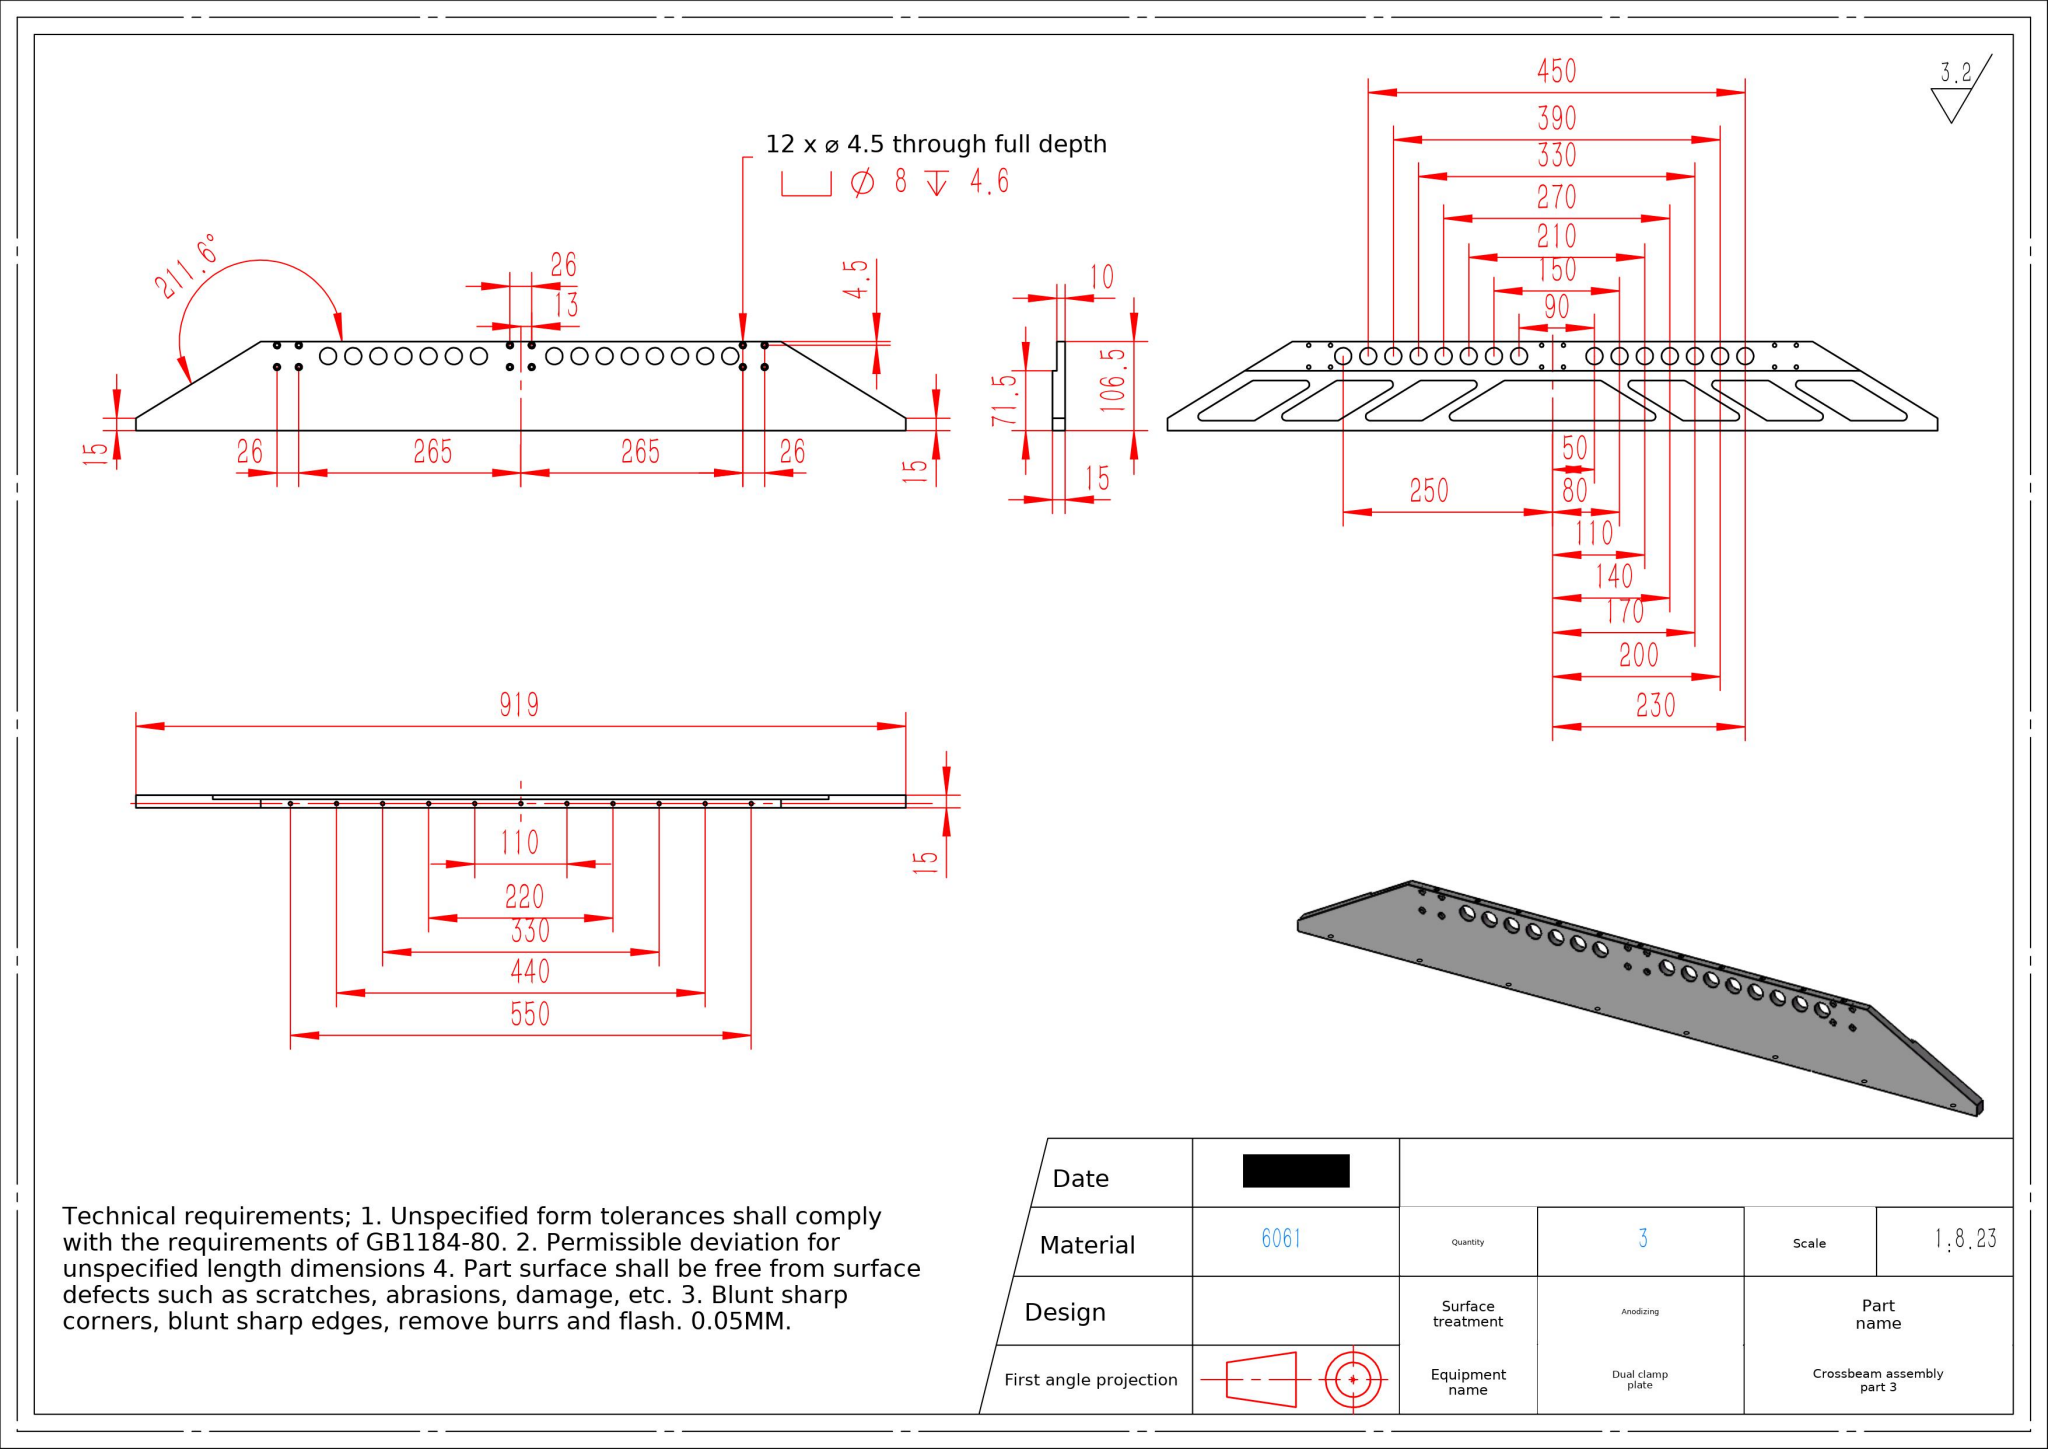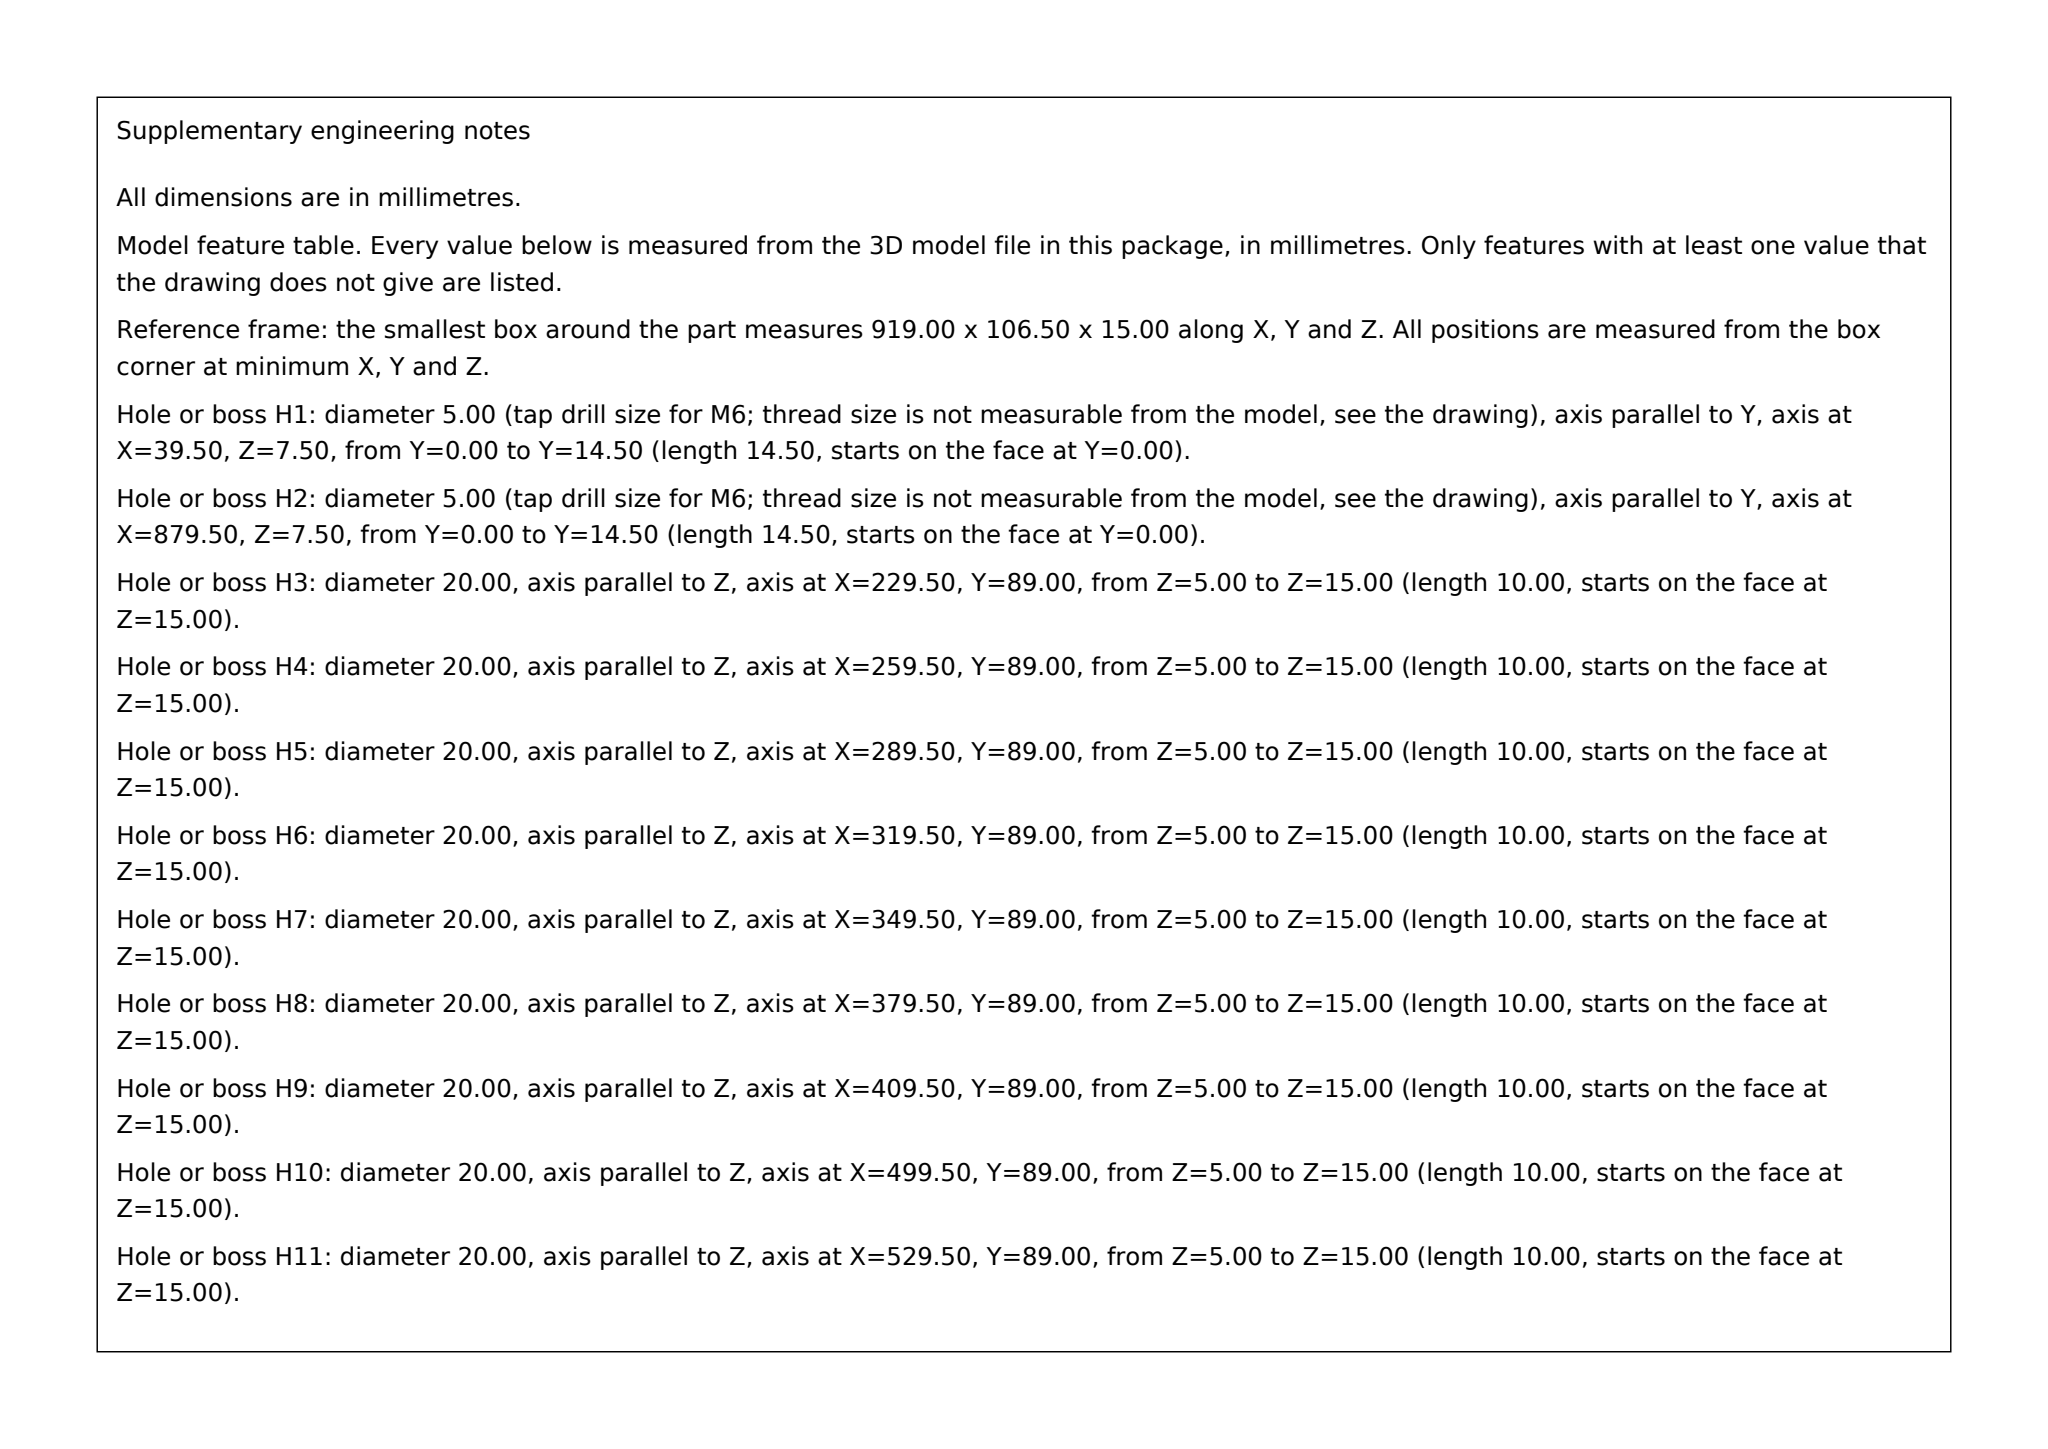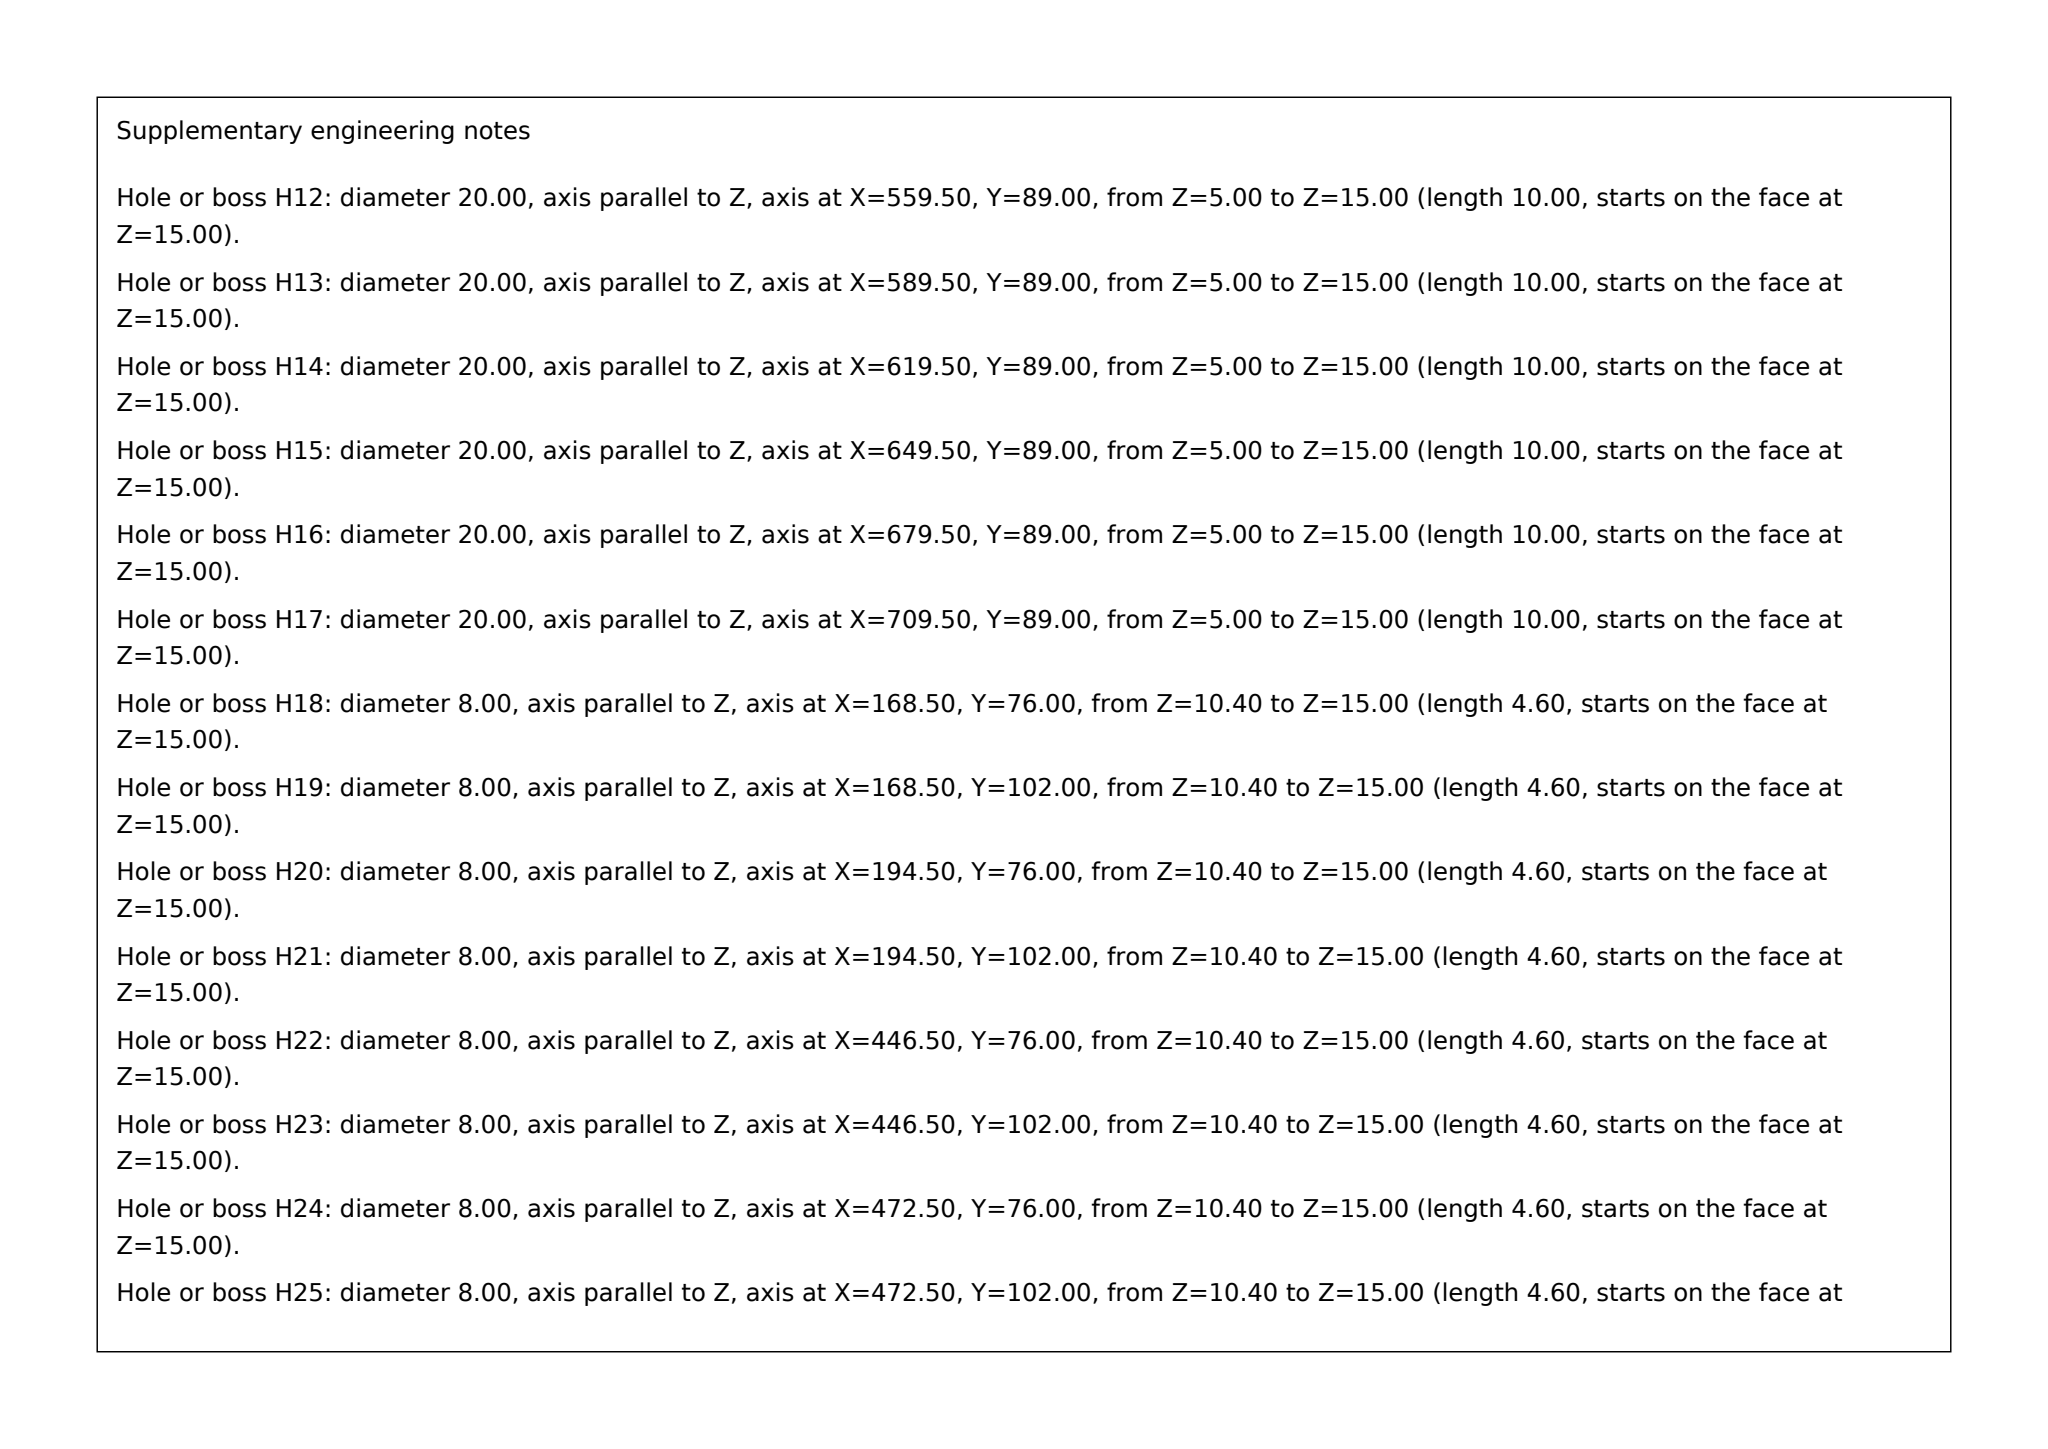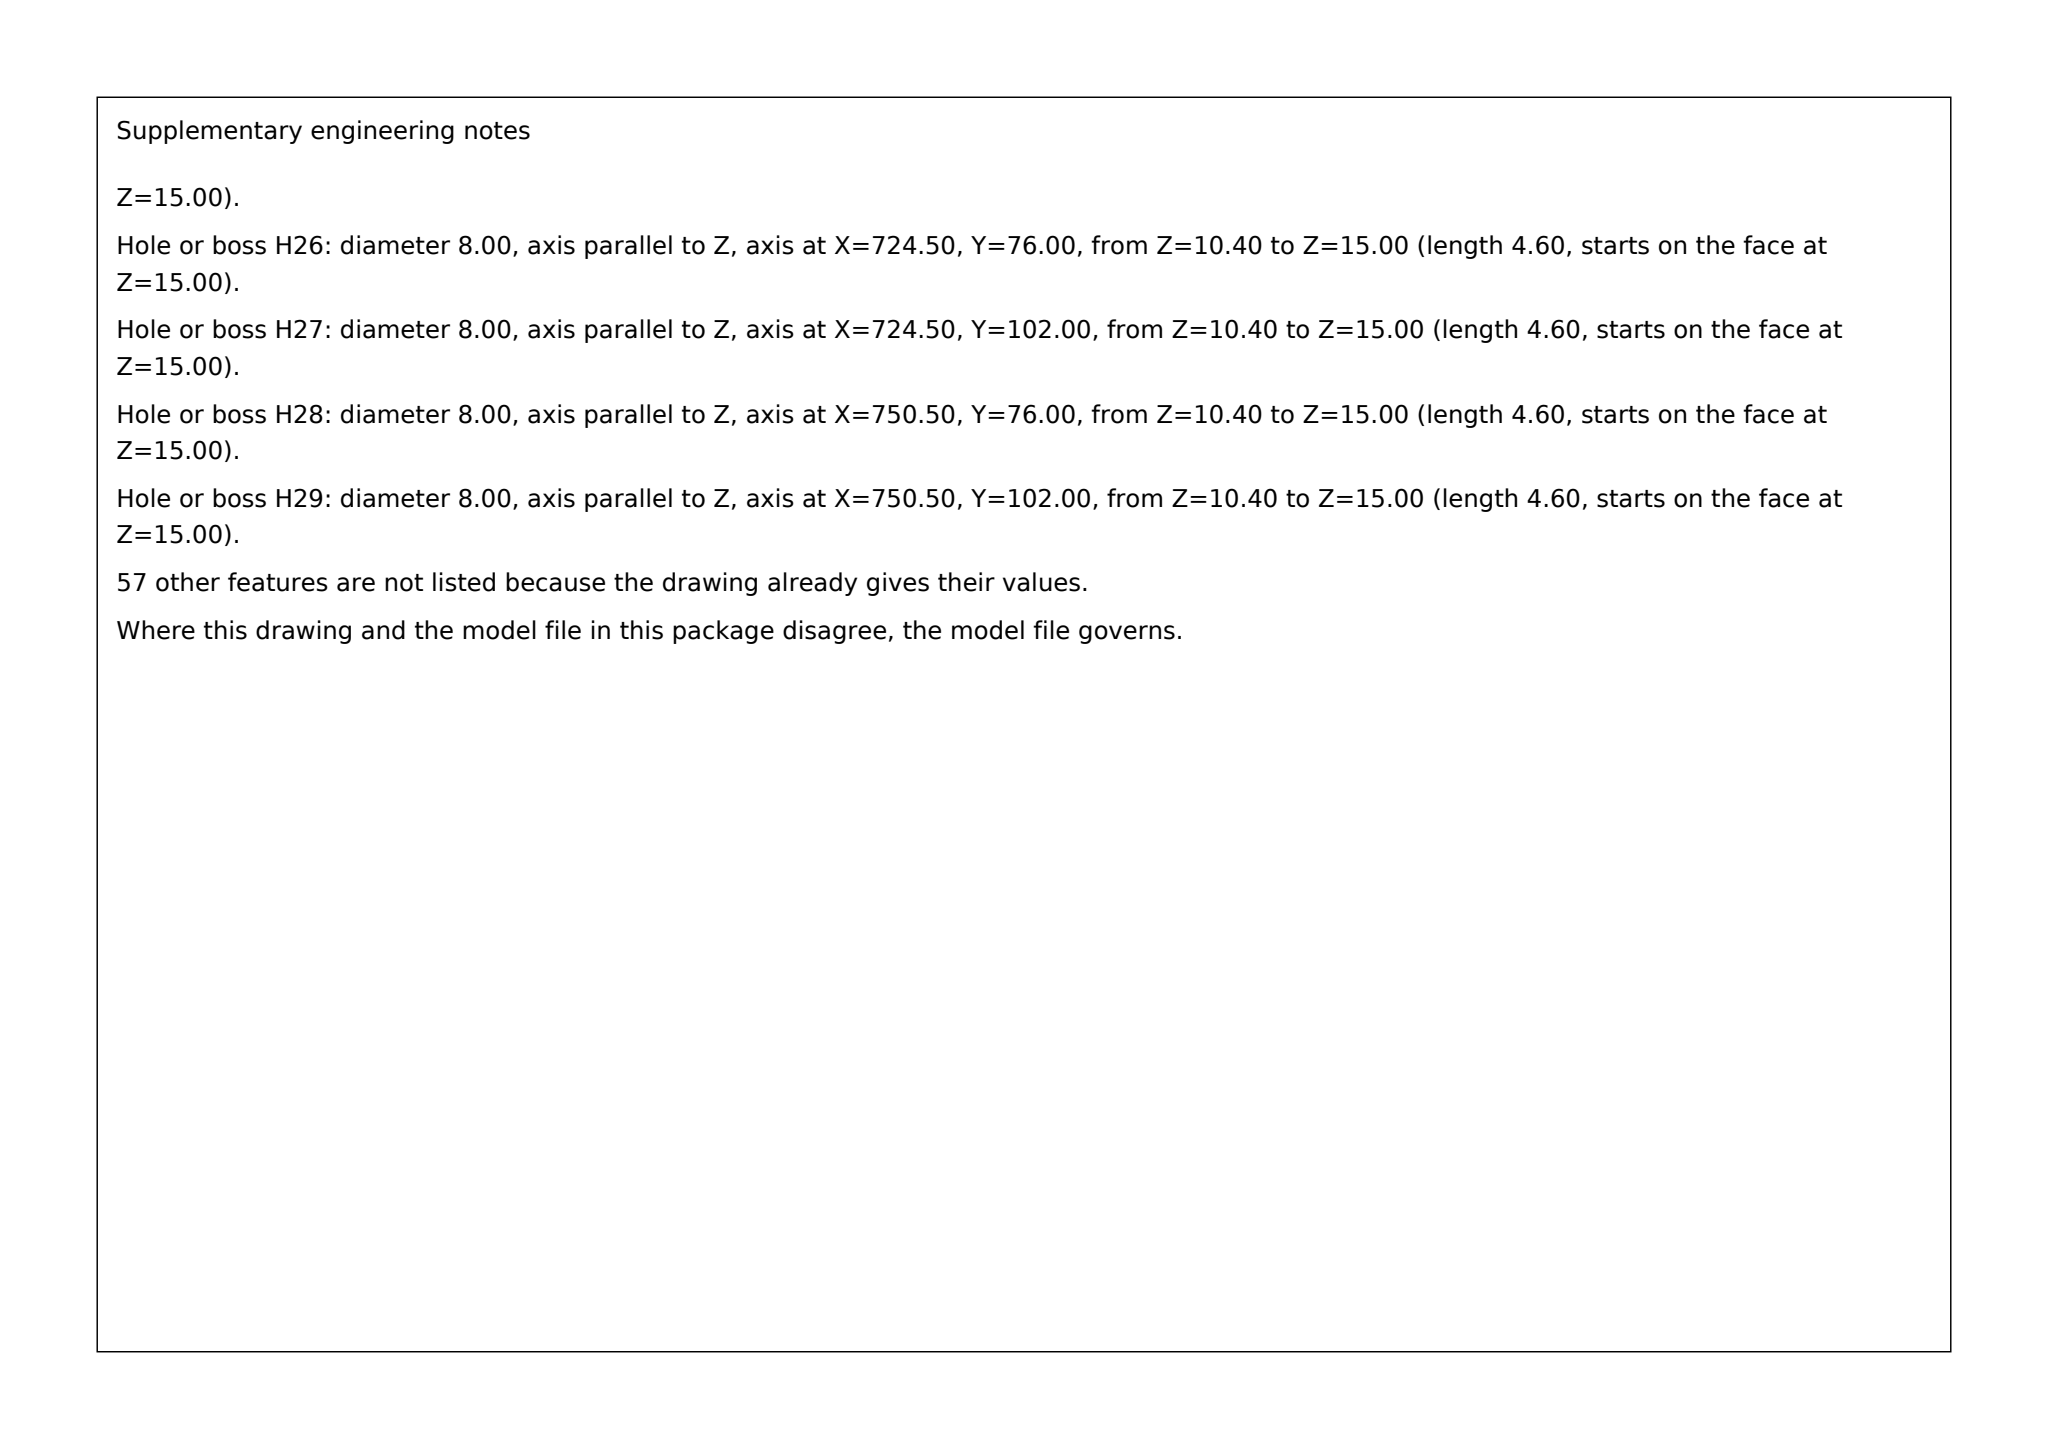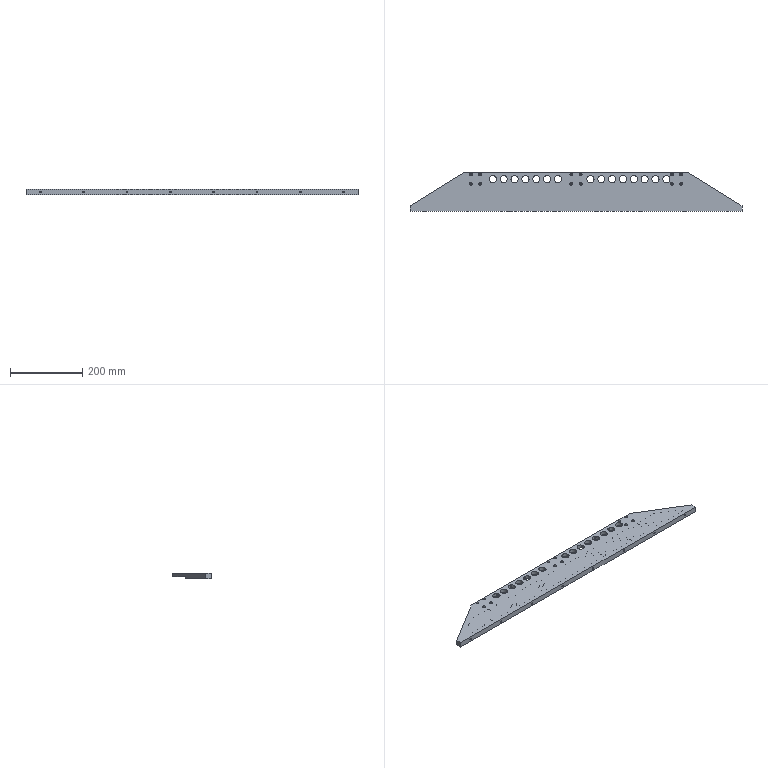Part | SolidWorks | mm | material 6061 | 1 solid | 222 faces | box 919 x 106.5 x 15 mm | volume 680585 mm3 | cylinder 151 | plane 57 | cone 14 | commonest cylinder face diameters 10 x35 20 x30 8 x24 4.5 x24 4.2 x22 5 x16